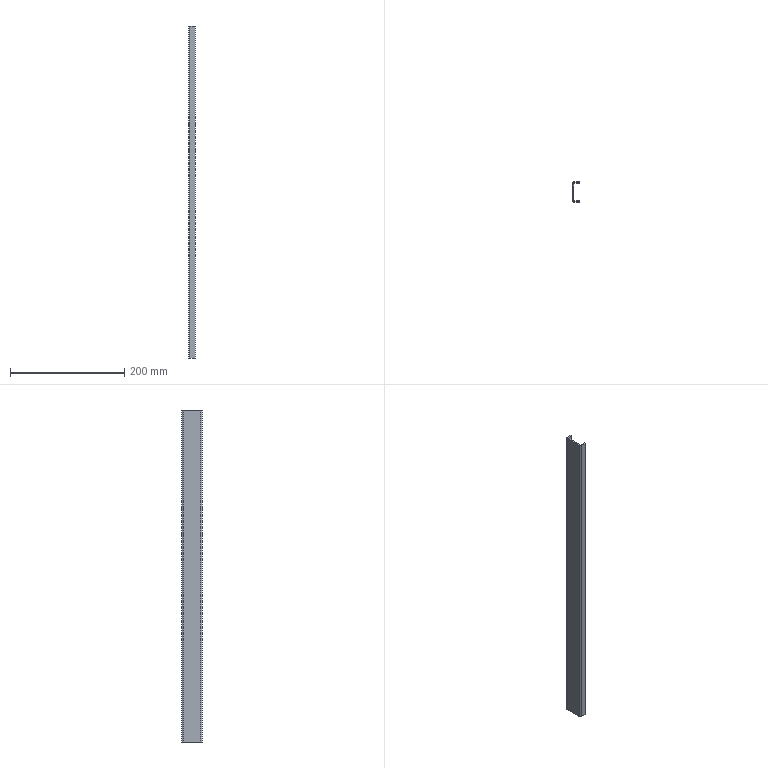Component | SolidWorks | PG50-06(BottomPlateWeldingDrawing)-1_BasePlateWeldment2(PG50-05-102-1 | 1 solid | 22 faces | box 12 x 35 x 580 mm | volume 62655 mm3 | plane 18 | cylinder 4 | commonest cylinder face diameters 4.3 x2 0.3 x2 | material AISI 1045 Steel, cold drawn
STEP:
#1=COLOUR_RGB('',0.7922,0.8196,0.9333);
#2=FILL_AREA_STYLE_COLOUR('',#1);
#3=FILL_AREA_STYLE('',(#2));
#4=SURFACE_STYLE_FILL_AREA(#3);
#5=SURFACE_SIDE_STYLE('',(#4));
#6=SURFACE_STYLE_USAGE(.BOTH.,#5);
#7=PRESENTATION_STYLE_ASSIGNMENT((#6));
#8=CARTESIAN_POINT('',(39.678,-0.2223,-11.417));
#9=VERTEX_POINT('',#8);
#10=CARTESIAN_POINT('',(39.678,-0.2223,11.417));
#11=VERTEX_POINT('',#10);
#12=CARTESIAN_POINT('',(39.678,-0.2223,-11.417));
#13=DIRECTION('',(-0.,0.,1.));
#14=VECTOR('',#13,39.37);
#15=LINE('',#12,#14);
#16=EDGE_CURVE('',#9,#11,#15,.T.);
#17=ORIENTED_EDGE('',*,*,#16,.T.);
#18=CARTESIAN_POINT('',(39.678,0.9864,11.417));
#19=VERTEX_POINT('',#18);
#20=CARTESIAN_POINT('',(39.678,-0.3069,11.417));
#21=DIRECTION('',(0.,-1.,0.));
#22=VECTOR('',#21,39.37);
#23=LINE('',#20,#22);
#24=EDGE_CURVE('',#19,#11,#23,.T.);
#25=ORIENTED_EDGE('',*,*,#24,.F.);
#26=CARTESIAN_POINT('',(39.678,0.9864,-11.417));
#27=VERTEX_POINT('',#26);
#28=CARTESIAN_POINT('',(39.678,0.9864,11.417));
#29=DIRECTION('',(-0.,-0.,-1.));
#30=VECTOR('',#29,39.37);
#31=LINE('',#28,#30);
#32=EDGE_CURVE('',#19,#27,#31,.T.);
#33=ORIENTED_EDGE('',*,*,#32,.T.);
#34=CARTESIAN_POINT('',(39.678,-0.3069,-11.417));
#35=DIRECTION('',(-0.,1.,-0.));
#36=VECTOR('',#35,39.37);
#37=LINE('',#34,#36);
#38=EDGE_CURVE('',#9,#27,#37,.T.);
#39=ORIENTED_EDGE('',*,*,#38,.F.);
#40=EDGE_LOOP('',(#17,#25,#33,#39));
#41=FACE_OUTER_BOUND('',#40,.T.);
#42=CARTESIAN_POINT('',(39.678,0.3821,-0.));
#43=DIRECTION('',(1.,0.,0.));
#44=DIRECTION('',(0.,-0.,-1.));
#45=AXIS2_PLACEMENT_3D('',#42,#43,#44);
#46=PLANE('',#45);
#47=ADVANCED_FACE('',(#41),#46,.F.);
#48=CARTESIAN_POINT('',(39.757,0.9864,11.417));
#49=VERTEX_POINT('',#48);
#50=CARTESIAN_POINT('',(39.757,-0.2223,11.417));
#51=VERTEX_POINT('',#50);
#52=CARTESIAN_POINT('',(39.757,-0.3069,11.417));
#53=DIRECTION('',(0.,-1.,0.));
#54=VECTOR('',#53,39.37);
#55=LINE('',#52,#54);
#56=EDGE_CURVE('',#49,#51,#55,.T.);
#57=ORIENTED_EDGE('',*,*,#56,.T.);
#58=CARTESIAN_POINT('',(39.757,-0.2223,-11.417));
#59=VERTEX_POINT('',#58);
#60=CARTESIAN_POINT('',(39.757,-0.2223,-11.417));
#61=DIRECTION('',(-0.,0.,1.));
#62=VECTOR('',#61,39.37);
#63=LINE('',#60,#62);
#64=EDGE_CURVE('',#59,#51,#63,.T.);
#65=ORIENTED_EDGE('',*,*,#64,.F.);
#66=CARTESIAN_POINT('',(39.757,0.9864,-11.417));
#67=VERTEX_POINT('',#66);
#68=CARTESIAN_POINT('',(39.757,-0.3069,-11.417));
#69=DIRECTION('',(-0.,1.,-0.));
#70=VECTOR('',#69,39.37);
#71=LINE('',#68,#70);
#72=EDGE_CURVE('',#59,#67,#71,.T.);
#73=ORIENTED_EDGE('',*,*,#72,.T.);
#74=CARTESIAN_POINT('',(39.757,0.9864,11.417));
#75=DIRECTION('',(-0.,-0.,-1.));
#76=VECTOR('',#75,39.37);
#77=LINE('',#74,#76);
#78=EDGE_CURVE('',#49,#67,#77,.T.);
#79=ORIENTED_EDGE('',*,*,#78,.F.);
#80=EDGE_LOOP('',(#57,#65,#73,#79));
#81=FACE_OUTER_BOUND('',#80,.T.);
#82=CARTESIAN_POINT('',(39.757,0.3821,-0.));
#83=DIRECTION('',(1.,0.,0.));
#84=DIRECTION('',(0.,-0.,-1.));
#85=AXIS2_PLACEMENT_3D('',#82,#83,#84);
#86=PLANE('',#85);
#87=ADVANCED_FACE('',(#81),#86,.T.);
#88=ORIENTED_EDGE('',*,*,#72,.F.);
#89=CARTESIAN_POINT('',(39.757,-0.2223,-11.417));
#90=DIRECTION('',(-1.,0.,-0.));
#91=VECTOR('',#90,39.37);
#92=LINE('',#89,#91);
#93=EDGE_CURVE('',#59,#9,#92,.T.);
#94=ORIENTED_EDGE('',*,*,#93,.T.);
#95=ORIENTED_EDGE('',*,*,#38,.T.);
#96=CARTESIAN_POINT('',(39.757,0.9864,-11.417));
#97=DIRECTION('',(-1.,-0.,-0.));
#98=VECTOR('',#97,39.37);
#99=LINE('',#96,#98);
#100=EDGE_CURVE('',#67,#27,#99,.T.);
#101=ORIENTED_EDGE('',*,*,#100,.F.);
#102=EDGE_LOOP('',(#88,#94,#95,#101));
#103=FACE_OUTER_BOUND('',#102,.T.);
#104=CARTESIAN_POINT('',(39.678,-0.3069,-11.417));
#105=DIRECTION('',(0.,-0.,-1.));
#106=DIRECTION('',(-1.,-0.,-0.));
#107=AXIS2_PLACEMENT_3D('',#104,#105,#106);
#108=PLANE('',#107);
#109=ADVANCED_FACE('',(#103),#108,.T.);
#110=CARTESIAN_POINT('',(39.757,-0.2223,11.417));
#111=DIRECTION('',(-1.,0.,-0.));
#112=VECTOR('',#111,39.37);
#113=LINE('',#110,#112);
#114=EDGE_CURVE('',#51,#11,#113,.T.);
#115=ORIENTED_EDGE('',*,*,#114,.F.);
#116=ORIENTED_EDGE('',*,*,#56,.F.);
#117=CARTESIAN_POINT('',(39.757,0.9864,11.417));
#118=DIRECTION('',(-1.,-0.,0.));
#119=VECTOR('',#118,39.37);
#120=LINE('',#117,#119);
#121=EDGE_CURVE('',#49,#19,#120,.T.);
#122=ORIENTED_EDGE('',*,*,#121,.T.);
#123=ORIENTED_EDGE('',*,*,#24,.T.);
#124=EDGE_LOOP('',(#115,#116,#122,#123));
#125=FACE_OUTER_BOUND('',#124,.T.);
#126=CARTESIAN_POINT('',(39.678,-0.3069,11.417));
#127=DIRECTION('',(-0.,0.,1.));
#128=DIRECTION('',(1.,0.,0.));
#129=AXIS2_PLACEMENT_3D('',#126,#127,#128);
#130=PLANE('',#129);
#131=ADVANCED_FACE('',(#125),#130,.T.);
#132=CARTESIAN_POINT('',(39.763,0.9923,-11.417));
#133=VERTEX_POINT('',#132);
#134=CARTESIAN_POINT('',(39.763,1.071,-11.417));
#135=VERTEX_POINT('',#134);
#136=CARTESIAN_POINT('',(39.763,1.071,-11.417));
#137=DIRECTION('',(-0.,1.,0.));
#138=VECTOR('',#137,39.37);
#139=LINE('',#136,#138);
#140=EDGE_CURVE('',#133,#135,#139,.T.);
#141=ORIENTED_EDGE('',*,*,#140,.F.);
#142=CARTESIAN_POINT('',(39.763,0.9864,-11.417));
#143=DIRECTION('',(-0.,-0.,-1.));
#144=DIRECTION('',(1.,0.,0.));
#145=AXIS2_PLACEMENT_3D('',#142,#143,#144);
#146=CIRCLE('',#145,0.005906);
#147=EDGE_CURVE('',#67,#133,#146,.T.);
#148=ORIENTED_EDGE('',*,*,#147,.F.);
#149=ORIENTED_EDGE('',*,*,#100,.T.);
#150=CARTESIAN_POINT('',(39.763,0.9864,-11.417));
#151=DIRECTION('',(-0.,-0.,-1.));
#152=DIRECTION('',(1.,0.,0.));
#153=AXIS2_PLACEMENT_3D('',#150,#151,#152);
#154=CIRCLE('',#153,0.08465);
#155=EDGE_CURVE('',#27,#135,#154,.T.);
#156=ORIENTED_EDGE('',*,*,#155,.T.);
#157=EDGE_LOOP('',(#141,#148,#149,#156));
#158=FACE_OUTER_BOUND('',#157,.T.);
#159=CARTESIAN_POINT('',(39.763,0.9864,-11.417));
#160=DIRECTION('',(-0.,-0.,-1.));
#161=DIRECTION('',(-1.,-0.,0.));
#162=AXIS2_PLACEMENT_3D('',#159,#160,#161);
#163=PLANE('',#162);
#164=ADVANCED_FACE('',(#158),#163,.T.);
#165=CARTESIAN_POINT('',(39.763,0.9923,11.417));
#166=VERTEX_POINT('',#165);
#167=CARTESIAN_POINT('',(39.763,0.9864,11.417));
#168=DIRECTION('',(0.,0.,1.));
#169=DIRECTION('',(1.,0.,0.));
#170=AXIS2_PLACEMENT_3D('',#167,#168,#169);
#171=CIRCLE('',#170,0.005906);
#172=EDGE_CURVE('',#166,#49,#171,.T.);
#173=ORIENTED_EDGE('',*,*,#172,.F.);
#174=CARTESIAN_POINT('',(39.763,1.071,11.417));
#175=VERTEX_POINT('',#174);
#176=CARTESIAN_POINT('',(39.763,0.9923,11.417));
#177=DIRECTION('',(-0.,1.,0.));
#178=VECTOR('',#177,39.37);
#179=LINE('',#176,#178);
#180=EDGE_CURVE('',#166,#175,#179,.T.);
#181=ORIENTED_EDGE('',*,*,#180,.T.);
#182=CARTESIAN_POINT('',(39.763,0.9864,11.417));
#183=DIRECTION('',(0.,0.,1.));
#184=DIRECTION('',(1.,0.,0.));
#185=AXIS2_PLACEMENT_3D('',#182,#183,#184);
#186=CIRCLE('',#185,0.08465);
#187=EDGE_CURVE('',#175,#19,#186,.T.);
#188=ORIENTED_EDGE('',*,*,#187,.T.);
#189=ORIENTED_EDGE('',*,*,#121,.F.);
#190=EDGE_LOOP('',(#173,#181,#188,#189));
#191=FACE_OUTER_BOUND('',#190,.T.);
#192=CARTESIAN_POINT('',(39.763,0.9864,11.417));
#193=DIRECTION('',(-0.,-0.,-1.));
#194=DIRECTION('',(-1.,-0.,0.));
#195=AXIS2_PLACEMENT_3D('',#192,#193,#194);
#196=PLANE('',#195);
#197=ADVANCED_FACE('',(#191),#196,.F.);
#198=ORIENTED_EDGE('',*,*,#32,.F.);
#199=ORIENTED_EDGE('',*,*,#187,.F.);
#200=CARTESIAN_POINT('',(39.763,1.071,-11.417));
#201=DIRECTION('',(-0.,0.,-1.));
#202=VECTOR('',#201,39.37);
#203=LINE('',#200,#202);
#204=EDGE_CURVE('',#175,#135,#203,.T.);
#205=ORIENTED_EDGE('',*,*,#204,.T.);
#206=ORIENTED_EDGE('',*,*,#155,.F.);
#207=EDGE_LOOP('',(#198,#199,#205,#206));
#208=FACE_OUTER_BOUND('',#207,.T.);
#209=CARTESIAN_POINT('',(39.763,0.9864,11.417));
#210=DIRECTION('',(0.,0.,1.));
#211=DIRECTION('',(0.,1.,0.));
#212=AXIS2_PLACEMENT_3D('',#209,#210,#211);
#213=CYLINDRICAL_SURFACE('',#212,0.08465);
#214=ADVANCED_FACE('',(#208),#213,.T.);
#215=ORIENTED_EDGE('',*,*,#78,.T.);
#216=ORIENTED_EDGE('',*,*,#147,.T.);
#217=CARTESIAN_POINT('',(39.763,0.9923,-11.417));
#218=DIRECTION('',(0.,-0.,1.));
#219=VECTOR('',#218,39.37);
#220=LINE('',#217,#219);
#221=EDGE_CURVE('',#133,#166,#220,.T.);
#222=ORIENTED_EDGE('',*,*,#221,.T.);
#223=ORIENTED_EDGE('',*,*,#172,.T.);
#224=EDGE_LOOP('',(#215,#216,#222,#223));
#225=FACE_OUTER_BOUND('',#224,.T.);
#226=CARTESIAN_POINT('',(39.763,0.9864,11.417));
#227=DIRECTION('',(0.,0.,1.));
#228=DIRECTION('',(0.,1.,0.));
#229=AXIS2_PLACEMENT_3D('',#226,#227,#228);
#230=CYLINDRICAL_SURFACE('',#229,0.005906);
#231=ADVANCED_FACE('',(#225),#230,.F.);
#232=ORIENTED_EDGE('',*,*,#140,.T.);
#233=CARTESIAN_POINT('',(40.15,1.071,-11.417));
#234=VERTEX_POINT('',#233);
#235=CARTESIAN_POINT('',(39.757,1.071,-11.417));
#236=DIRECTION('',(-1.,-0.,-0.));
#237=VECTOR('',#236,39.37);
#238=LINE('',#235,#237);
#239=EDGE_CURVE('',#234,#135,#238,.T.);
#240=ORIENTED_EDGE('',*,*,#239,.F.);
#241=CARTESIAN_POINT('',(40.15,0.9923,-11.417));
#242=VERTEX_POINT('',#241);
#243=CARTESIAN_POINT('',(40.15,1.071,-11.417));
#244=DIRECTION('',(0.,-1.,-0.));
#245=VECTOR('',#244,39.37);
#246=LINE('',#243,#245);
#247=EDGE_CURVE('',#234,#242,#246,.T.);
#248=ORIENTED_EDGE('',*,*,#247,.T.);
#249=CARTESIAN_POINT('',(39.757,0.9923,-11.417));
#250=DIRECTION('',(-1.,-0.,-0.));
#251=VECTOR('',#250,39.37);
#252=LINE('',#249,#251);
#253=EDGE_CURVE('',#242,#133,#252,.T.);
#254=ORIENTED_EDGE('',*,*,#253,.T.);
#255=EDGE_LOOP('',(#232,#240,#248,#254));
#256=FACE_OUTER_BOUND('',#255,.T.);
#257=CARTESIAN_POINT('',(39.757,1.071,-11.417));
#258=DIRECTION('',(-0.,-0.,1.));
#259=DIRECTION('',(0.,-1.,-0.));
#260=AXIS2_PLACEMENT_3D('',#257,#258,#259);
#261=PLANE('',#260);
#262=ADVANCED_FACE('',(#256),#261,.F.);
#263=ORIENTED_EDGE('',*,*,#180,.F.);
#264=CARTESIAN_POINT('',(40.15,0.9923,11.417));
#265=VERTEX_POINT('',#264);
#266=CARTESIAN_POINT('',(40.15,0.9923,11.417));
#267=DIRECTION('',(1.,0.,0.));
#268=VECTOR('',#267,39.37);
#269=LINE('',#266,#268);
#270=EDGE_CURVE('',#166,#265,#269,.T.);
#271=ORIENTED_EDGE('',*,*,#270,.T.);
#272=CARTESIAN_POINT('',(40.15,1.071,11.417));
#273=VERTEX_POINT('',#272);
#274=CARTESIAN_POINT('',(40.15,1.071,11.417));
#275=DIRECTION('',(0.,-1.,-0.));
#276=VECTOR('',#275,39.37);
#277=LINE('',#274,#276);
#278=EDGE_CURVE('',#273,#265,#277,.T.);
#279=ORIENTED_EDGE('',*,*,#278,.F.);
#280=CARTESIAN_POINT('',(39.757,1.071,11.417));
#281=DIRECTION('',(1.,0.,0.));
#282=VECTOR('',#281,39.37);
#283=LINE('',#280,#282);
#284=EDGE_CURVE('',#175,#273,#283,.T.);
#285=ORIENTED_EDGE('',*,*,#284,.F.);
#286=EDGE_LOOP('',(#263,#271,#279,#285));
#287=FACE_OUTER_BOUND('',#286,.T.);
#288=CARTESIAN_POINT('',(40.15,1.071,11.417));
#289=DIRECTION('',(0.,0.,-1.));
#290=DIRECTION('',(-0.,1.,0.));
#291=AXIS2_PLACEMENT_3D('',#288,#289,#290);
#292=PLANE('',#291);
#293=ADVANCED_FACE('',(#287),#292,.F.);
#294=ORIENTED_EDGE('',*,*,#204,.F.);
#295=ORIENTED_EDGE('',*,*,#284,.T.);
#296=CARTESIAN_POINT('',(40.15,1.071,-0.));
#297=DIRECTION('',(0.,0.,-1.));
#298=VECTOR('',#297,39.37);
#299=LINE('',#296,#298);
#300=EDGE_CURVE('',#273,#234,#299,.T.);
#301=ORIENTED_EDGE('',*,*,#300,.T.);
#302=ORIENTED_EDGE('',*,*,#239,.T.);
#303=EDGE_LOOP('',(#294,#295,#301,#302));
#304=FACE_OUTER_BOUND('',#303,.T.);
#305=CARTESIAN_POINT('',(39.757,1.071,-0.));
#306=DIRECTION('',(0.,-1.,-0.));
#307=DIRECTION('',(-1.,-0.,-0.));
#308=AXIS2_PLACEMENT_3D('',#305,#306,#307);
#309=PLANE('',#308);
#310=ADVANCED_FACE('',(#304),#309,.F.);
#311=ORIENTED_EDGE('',*,*,#270,.F.);
#312=ORIENTED_EDGE('',*,*,#221,.F.);
#313=ORIENTED_EDGE('',*,*,#253,.F.);
#314=CARTESIAN_POINT('',(40.15,0.9923,-11.417));
#315=DIRECTION('',(0.,0.,-1.));
#316=VECTOR('',#315,39.37);
#317=LINE('',#314,#316);
#318=EDGE_CURVE('',#265,#242,#317,.T.);
#319=ORIENTED_EDGE('',*,*,#318,.F.);
#320=EDGE_LOOP('',(#311,#312,#313,#319));
#321=FACE_OUTER_BOUND('',#320,.T.);
#322=CARTESIAN_POINT('',(39.757,0.9923,-0.));
#323=DIRECTION('',(0.,-1.,-0.));
#324=DIRECTION('',(-1.,-0.,-0.));
#325=AXIS2_PLACEMENT_3D('',#322,#323,#324);
#326=PLANE('',#325);
#327=ADVANCED_FACE('',(#321),#326,.T.);
#328=ORIENTED_EDGE('',*,*,#318,.T.);
#329=ORIENTED_EDGE('',*,*,#247,.F.);
#330=ORIENTED_EDGE('',*,*,#300,.F.);
#331=ORIENTED_EDGE('',*,*,#278,.T.);
#332=EDGE_LOOP('',(#328,#329,#330,#331));
#333=FACE_OUTER_BOUND('',#332,.T.);
#334=CARTESIAN_POINT('',(40.15,1.071,-11.417));
#335=DIRECTION('',(-1.,-0.,-0.));
#336=DIRECTION('',(-0.,1.,-0.));
#337=AXIS2_PLACEMENT_3D('',#334,#335,#336);
#338=PLANE('',#337);
#339=ADVANCED_FACE('',(#333),#338,.F.);
#340=CARTESIAN_POINT('',(39.763,-0.2282,11.417));
#341=VERTEX_POINT('',#340);
#342=CARTESIAN_POINT('',(39.763,-0.3069,11.417));
#343=VERTEX_POINT('',#342);
#344=CARTESIAN_POINT('',(39.763,-0.3069,11.417));
#345=DIRECTION('',(-0.,-1.,-0.));
#346=VECTOR('',#345,39.37);
#347=LINE('',#344,#346);
#348=EDGE_CURVE('',#341,#343,#347,.T.);
#349=ORIENTED_EDGE('',*,*,#348,.F.);
#350=CARTESIAN_POINT('',(39.763,-0.2223,11.417));
#351=DIRECTION('',(-0.,0.,1.));
#352=DIRECTION('',(-1.,0.,0.));
#353=AXIS2_PLACEMENT_3D('',#350,#351,#352);
#354=CIRCLE('',#353,0.005906);
#355=EDGE_CURVE('',#51,#341,#354,.T.);
#356=ORIENTED_EDGE('',*,*,#355,.F.);
#357=ORIENTED_EDGE('',*,*,#114,.T.);
#358=CARTESIAN_POINT('',(39.763,-0.2223,11.417));
#359=DIRECTION('',(-0.,0.,1.));
#360=DIRECTION('',(-1.,-0.,0.));
#361=AXIS2_PLACEMENT_3D('',#358,#359,#360);
#362=CIRCLE('',#361,0.08465);
#363=EDGE_CURVE('',#11,#343,#362,.T.);
#364=ORIENTED_EDGE('',*,*,#363,.T.);
#365=EDGE_LOOP('',(#349,#356,#357,#364));
#366=FACE_OUTER_BOUND('',#365,.T.);
#367=CARTESIAN_POINT('',(39.763,-0.2223,11.417));
#368=DIRECTION('',(-0.,0.,1.));
#369=DIRECTION('',(1.,0.,0.));
#370=AXIS2_PLACEMENT_3D('',#367,#368,#369);
#371=PLANE('',#370);
#372=ADVANCED_FACE('',(#366),#371,.T.);
#373=CARTESIAN_POINT('',(39.763,-0.2282,-11.417));
#374=VERTEX_POINT('',#373);
#375=CARTESIAN_POINT('',(39.763,-0.2223,-11.417));
#376=DIRECTION('',(0.,-0.,-1.));
#377=DIRECTION('',(-1.,-0.,0.));
#378=AXIS2_PLACEMENT_3D('',#375,#376,#377);
#379=CIRCLE('',#378,0.005906);
#380=EDGE_CURVE('',#374,#59,#379,.T.);
#381=ORIENTED_EDGE('',*,*,#380,.F.);
#382=CARTESIAN_POINT('',(39.763,-0.3069,-11.417));
#383=VERTEX_POINT('',#382);
#384=CARTESIAN_POINT('',(39.763,-0.2282,-11.417));
#385=DIRECTION('',(-0.,-1.,-0.));
#386=VECTOR('',#385,39.37);
#387=LINE('',#384,#386);
#388=EDGE_CURVE('',#374,#383,#387,.T.);
#389=ORIENTED_EDGE('',*,*,#388,.T.);
#390=CARTESIAN_POINT('',(39.763,-0.2223,-11.417));
#391=DIRECTION('',(0.,-0.,-1.));
#392=DIRECTION('',(-1.,-0.,0.));
#393=AXIS2_PLACEMENT_3D('',#390,#391,#392);
#394=CIRCLE('',#393,0.08465);
#395=EDGE_CURVE('',#383,#9,#394,.T.);
#396=ORIENTED_EDGE('',*,*,#395,.T.);
#397=ORIENTED_EDGE('',*,*,#93,.F.);
#398=EDGE_LOOP('',(#381,#389,#396,#397));
#399=FACE_OUTER_BOUND('',#398,.T.);
#400=CARTESIAN_POINT('',(39.763,-0.2223,-11.417));
#401=DIRECTION('',(-0.,0.,1.));
#402=DIRECTION('',(1.,0.,0.));
#403=AXIS2_PLACEMENT_3D('',#400,#401,#402);
#404=PLANE('',#403);
#405=ADVANCED_FACE('',(#399),#404,.F.);
#406=ORIENTED_EDGE('',*,*,#16,.F.);
#407=ORIENTED_EDGE('',*,*,#395,.F.);
#408=CARTESIAN_POINT('',(39.763,-0.3069,11.417));
#409=DIRECTION('',(-0.,-0.,1.));
#410=VECTOR('',#409,39.37);
#411=LINE('',#408,#410);
#412=EDGE_CURVE('',#383,#343,#411,.T.);
#413=ORIENTED_EDGE('',*,*,#412,.T.);
#414=ORIENTED_EDGE('',*,*,#363,.F.);
#415=EDGE_LOOP('',(#406,#407,#413,#414));
#416=FACE_OUTER_BOUND('',#415,.T.);
#417=CARTESIAN_POINT('',(39.763,-0.2223,-11.417));
#418=DIRECTION('',(0.,-0.,-1.));
#419=DIRECTION('',(0.,-1.,0.));
#420=AXIS2_PLACEMENT_3D('',#417,#418,#419);
#421=CYLINDRICAL_SURFACE('',#420,0.08465);
#422=ADVANCED_FACE('',(#416),#421,.T.);
#423=ORIENTED_EDGE('',*,*,#64,.T.);
#424=ORIENTED_EDGE('',*,*,#355,.T.);
#425=CARTESIAN_POINT('',(39.763,-0.2282,11.417));
#426=DIRECTION('',(0.,0.,-1.));
#427=VECTOR('',#426,39.37);
#428=LINE('',#425,#427);
#429=EDGE_CURVE('',#341,#374,#428,.T.);
#430=ORIENTED_EDGE('',*,*,#429,.T.);
#431=ORIENTED_EDGE('',*,*,#380,.T.);
#432=EDGE_LOOP('',(#423,#424,#430,#431));
#433=FACE_OUTER_BOUND('',#432,.T.);
#434=CARTESIAN_POINT('',(39.763,-0.2223,-11.417));
#435=DIRECTION('',(0.,-0.,-1.));
#436=DIRECTION('',(0.,-1.,0.));
#437=AXIS2_PLACEMENT_3D('',#434,#435,#436);
#438=CYLINDRICAL_SURFACE('',#437,0.005906);
#439=ADVANCED_FACE('',(#433),#438,.F.);
#440=ORIENTED_EDGE('',*,*,#348,.T.);
#441=CARTESIAN_POINT('',(40.15,-0.3069,11.417));
#442=VERTEX_POINT('',#441);
#443=CARTESIAN_POINT('',(39.757,-0.3069,11.417));
#444=DIRECTION('',(-1.,0.,-0.));
#445=VECTOR('',#444,39.37);
#446=LINE('',#443,#445);
#447=EDGE_CURVE('',#442,#343,#446,.T.);
#448=ORIENTED_EDGE('',*,*,#447,.F.);
#449=CARTESIAN_POINT('',(40.15,-0.2282,11.417));
#450=VERTEX_POINT('',#449);
#451=CARTESIAN_POINT('',(40.15,-0.3069,11.417));
#452=DIRECTION('',(0.,1.,0.));
#453=VECTOR('',#452,39.37);
#454=LINE('',#451,#453);
#455=EDGE_CURVE('',#442,#450,#454,.T.);
#456=ORIENTED_EDGE('',*,*,#455,.T.);
#457=CARTESIAN_POINT('',(39.757,-0.2282,11.417));
#458=DIRECTION('',(-1.,0.,-0.));
#459=VECTOR('',#458,39.37);
#460=LINE('',#457,#459);
#461=EDGE_CURVE('',#450,#341,#460,.T.);
#462=ORIENTED_EDGE('',*,*,#461,.T.);
#463=EDGE_LOOP('',(#440,#448,#456,#462));
#464=FACE_OUTER_BOUND('',#463,.T.);
#465=CARTESIAN_POINT('',(39.757,-0.3069,11.417));
#466=DIRECTION('',(0.,0.,-1.));
#467=DIRECTION('',(-0.,1.,0.));
#468=AXIS2_PLACEMENT_3D('',#465,#466,#467);
#469=PLANE('',#468);
#470=ADVANCED_FACE('',(#464),#469,.F.);
#471=ORIENTED_EDGE('',*,*,#388,.F.);
#472=CARTESIAN_POINT('',(40.15,-0.2282,-11.417));
#473=VERTEX_POINT('',#472);
#474=CARTESIAN_POINT('',(40.15,-0.2282,-11.417));
#475=DIRECTION('',(1.,-0.,0.));
#476=VECTOR('',#475,39.37);
#477=LINE('',#474,#476);
#478=EDGE_CURVE('',#374,#473,#477,.T.);
#479=ORIENTED_EDGE('',*,*,#478,.T.);
#480=CARTESIAN_POINT('',(40.15,-0.3069,-11.417));
#481=VERTEX_POINT('',#480);
#482=CARTESIAN_POINT('',(40.15,-0.3069,-11.417));
#483=DIRECTION('',(0.,1.,0.));
#484=VECTOR('',#483,39.37);
#485=LINE('',#482,#484);
#486=EDGE_CURVE('',#481,#473,#485,.T.);
#487=ORIENTED_EDGE('',*,*,#486,.F.);
#488=CARTESIAN_POINT('',(39.757,-0.3069,-11.417));
#489=DIRECTION('',(1.,-0.,0.));
#490=VECTOR('',#489,39.37);
#491=LINE('',#488,#490);
#492=EDGE_CURVE('',#383,#481,#491,.T.);
#493=ORIENTED_EDGE('',*,*,#492,.F.);
#494=EDGE_LOOP('',(#471,#479,#487,#493));
#495=FACE_OUTER_BOUND('',#494,.T.);
#496=CARTESIAN_POINT('',(40.15,-0.3069,-11.417));
#497=DIRECTION('',(-0.,-0.,1.));
#498=DIRECTION('',(0.,-1.,-0.));
#499=AXIS2_PLACEMENT_3D('',#496,#497,#498);
#500=PLANE('',#499);
#501=ADVANCED_FACE('',(#495),#500,.F.);
#502=ORIENTED_EDGE('',*,*,#412,.F.);
#503=ORIENTED_EDGE('',*,*,#492,.T.);
#504=CARTESIAN_POINT('',(40.15,-0.3069,-0.));
#505=DIRECTION('',(-0.,-0.,1.));
#506=VECTOR('',#505,39.37);
#507=LINE('',#504,#506);
#508=EDGE_CURVE('',#481,#442,#507,.T.);
#509=ORIENTED_EDGE('',*,*,#508,.T.);
#510=ORIENTED_EDGE('',*,*,#447,.T.);
#511=EDGE_LOOP('',(#502,#503,#509,#510));
#512=FACE_OUTER_BOUND('',#511,.T.);
#513=CARTESIAN_POINT('',(39.757,-0.3069,-0.));
#514=DIRECTION('',(0.,1.,0.));
#515=DIRECTION('',(1.,-0.,0.));
#516=AXIS2_PLACEMENT_3D('',#513,#514,#515);
#517=PLANE('',#516);
#518=ADVANCED_FACE('',(#512),#517,.F.);
#519=ORIENTED_EDGE('',*,*,#478,.F.);
#520=ORIENTED_EDGE('',*,*,#429,.F.);
#521=ORIENTED_EDGE('',*,*,#461,.F.);
#522=CARTESIAN_POINT('',(40.15,-0.2282,11.417));
#523=DIRECTION('',(-0.,-0.,1.));
#524=VECTOR('',#523,39.37);
#525=LINE('',#522,#524);
#526=EDGE_CURVE('',#473,#450,#525,.T.);
#527=ORIENTED_EDGE('',*,*,#526,.F.);
#528=EDGE_LOOP('',(#519,#520,#521,#527));
#529=FACE_OUTER_BOUND('',#528,.T.);
#530=CARTESIAN_POINT('',(39.757,-0.2282,-0.));
#531=DIRECTION('',(0.,1.,0.));
#532=DIRECTION('',(1.,-0.,0.));
#533=AXIS2_PLACEMENT_3D('',#530,#531,#532);
#534=PLANE('',#533);
#535=ADVANCED_FACE('',(#529),#534,.T.);
#536=ORIENTED_EDGE('',*,*,#526,.T.);
#537=ORIENTED_EDGE('',*,*,#455,.F.);
#538=ORIENTED_EDGE('',*,*,#508,.F.);
#539=ORIENTED_EDGE('',*,*,#486,.T.);
#540=EDGE_LOOP('',(#536,#537,#538,#539));
#541=FACE_OUTER_BOUND('',#540,.T.);
#542=CARTESIAN_POINT('',(40.15,-0.3069,11.417));
#543=DIRECTION('',(-1.,0.,-0.));
#544=DIRECTION('',(0.,1.,-0.));
#545=AXIS2_PLACEMENT_3D('',#542,#543,#544);
#546=PLANE('',#545);
#547=ADVANCED_FACE('',(#541),#546,.F.);
#548=CLOSED_SHELL('',(#47,#87,#109,#131,#164,#197,#214,#231,#262,#293,#310,#327,#339,#372,#405,#422,#439,#470,#501,#518,#535,#547));
#549=MANIFOLD_SOLID_BREP('',#548);
#550=STYLED_ITEM('',(#7),#549);
#551=(LENGTH_UNIT()NAMED_UNIT(*)SI_UNIT($,.METRE.));
#552=LENGTH_MEASURE_WITH_UNIT(LENGTH_MEASURE(0.0254),#551);
#553=DIMENSIONAL_EXPONENTS(1.,0.,0.,0.,0.,0.,0.);
#554=(CONVERSION_BASED_UNIT('',#552)LENGTH_UNIT()NAMED_UNIT(#553));
#555=UNCERTAINTY_MEASURE_WITH_UNIT(LENGTH_MEASURE(0.00001),#554,'','');
#556=(NAMED_UNIT(*)PLANE_ANGLE_UNIT()SI_UNIT($,.RADIAN.));
#557=(NAMED_UNIT(*)SI_UNIT($,.STERADIAN.)SOLID_ANGLE_UNIT());
#558=(GEOMETRIC_REPRESENTATION_CONTEXT(3)GLOBAL_UNCERTAINTY_ASSIGNED_CONTEXT((#555))GLOBAL_UNIT_ASSIGNED_CONTEXT((#554,#556,#557))REPRESENTATION_CONTEXT('',''));
#559=MECHANICAL_DESIGN_GEOMETRIC_PRESENTATION_REPRESENTATION('',(#550),#558);
#560=CARTESIAN_POINT('',(0.,0.,0.));
#561=DIRECTION('',(0.,0.,1.));
#562=DIRECTION('',(1.,0.,0.));
#563=AXIS2_PLACEMENT_3D('',#560,#561,#562);
#564=(LENGTH_UNIT()NAMED_UNIT(*)SI_UNIT($,.METRE.));
#565=LENGTH_MEASURE_WITH_UNIT(LENGTH_MEASURE(0.0254),#564);
#566=DIMENSIONAL_EXPONENTS(1.,0.,0.,0.,0.,0.,0.);
#567=(CONVERSION_BASED_UNIT('',#565)LENGTH_UNIT()NAMED_UNIT(#566));
#568=UNCERTAINTY_MEASURE_WITH_UNIT(LENGTH_MEASURE(0.00001),#567,'','');
#569=(NAMED_UNIT(*)PLANE_ANGLE_UNIT()SI_UNIT($,.RADIAN.));
#570=(NAMED_UNIT(*)SI_UNIT($,.STERADIAN.)SOLID_ANGLE_UNIT());
#571=(GEOMETRIC_REPRESENTATION_CONTEXT(3)GLOBAL_UNCERTAINTY_ASSIGNED_CONTEXT((#568))GLOBAL_UNIT_ASSIGNED_CONTEXT((#567,#569,#570))REPRESENTATION_CONTEXT('',''));
#572=ADVANCED_BREP_SHAPE_REPRESENTATION('',(#549,#563),#571);
#573=PRESENTATION_LAYER_ASSIGNMENT('','',(#550));